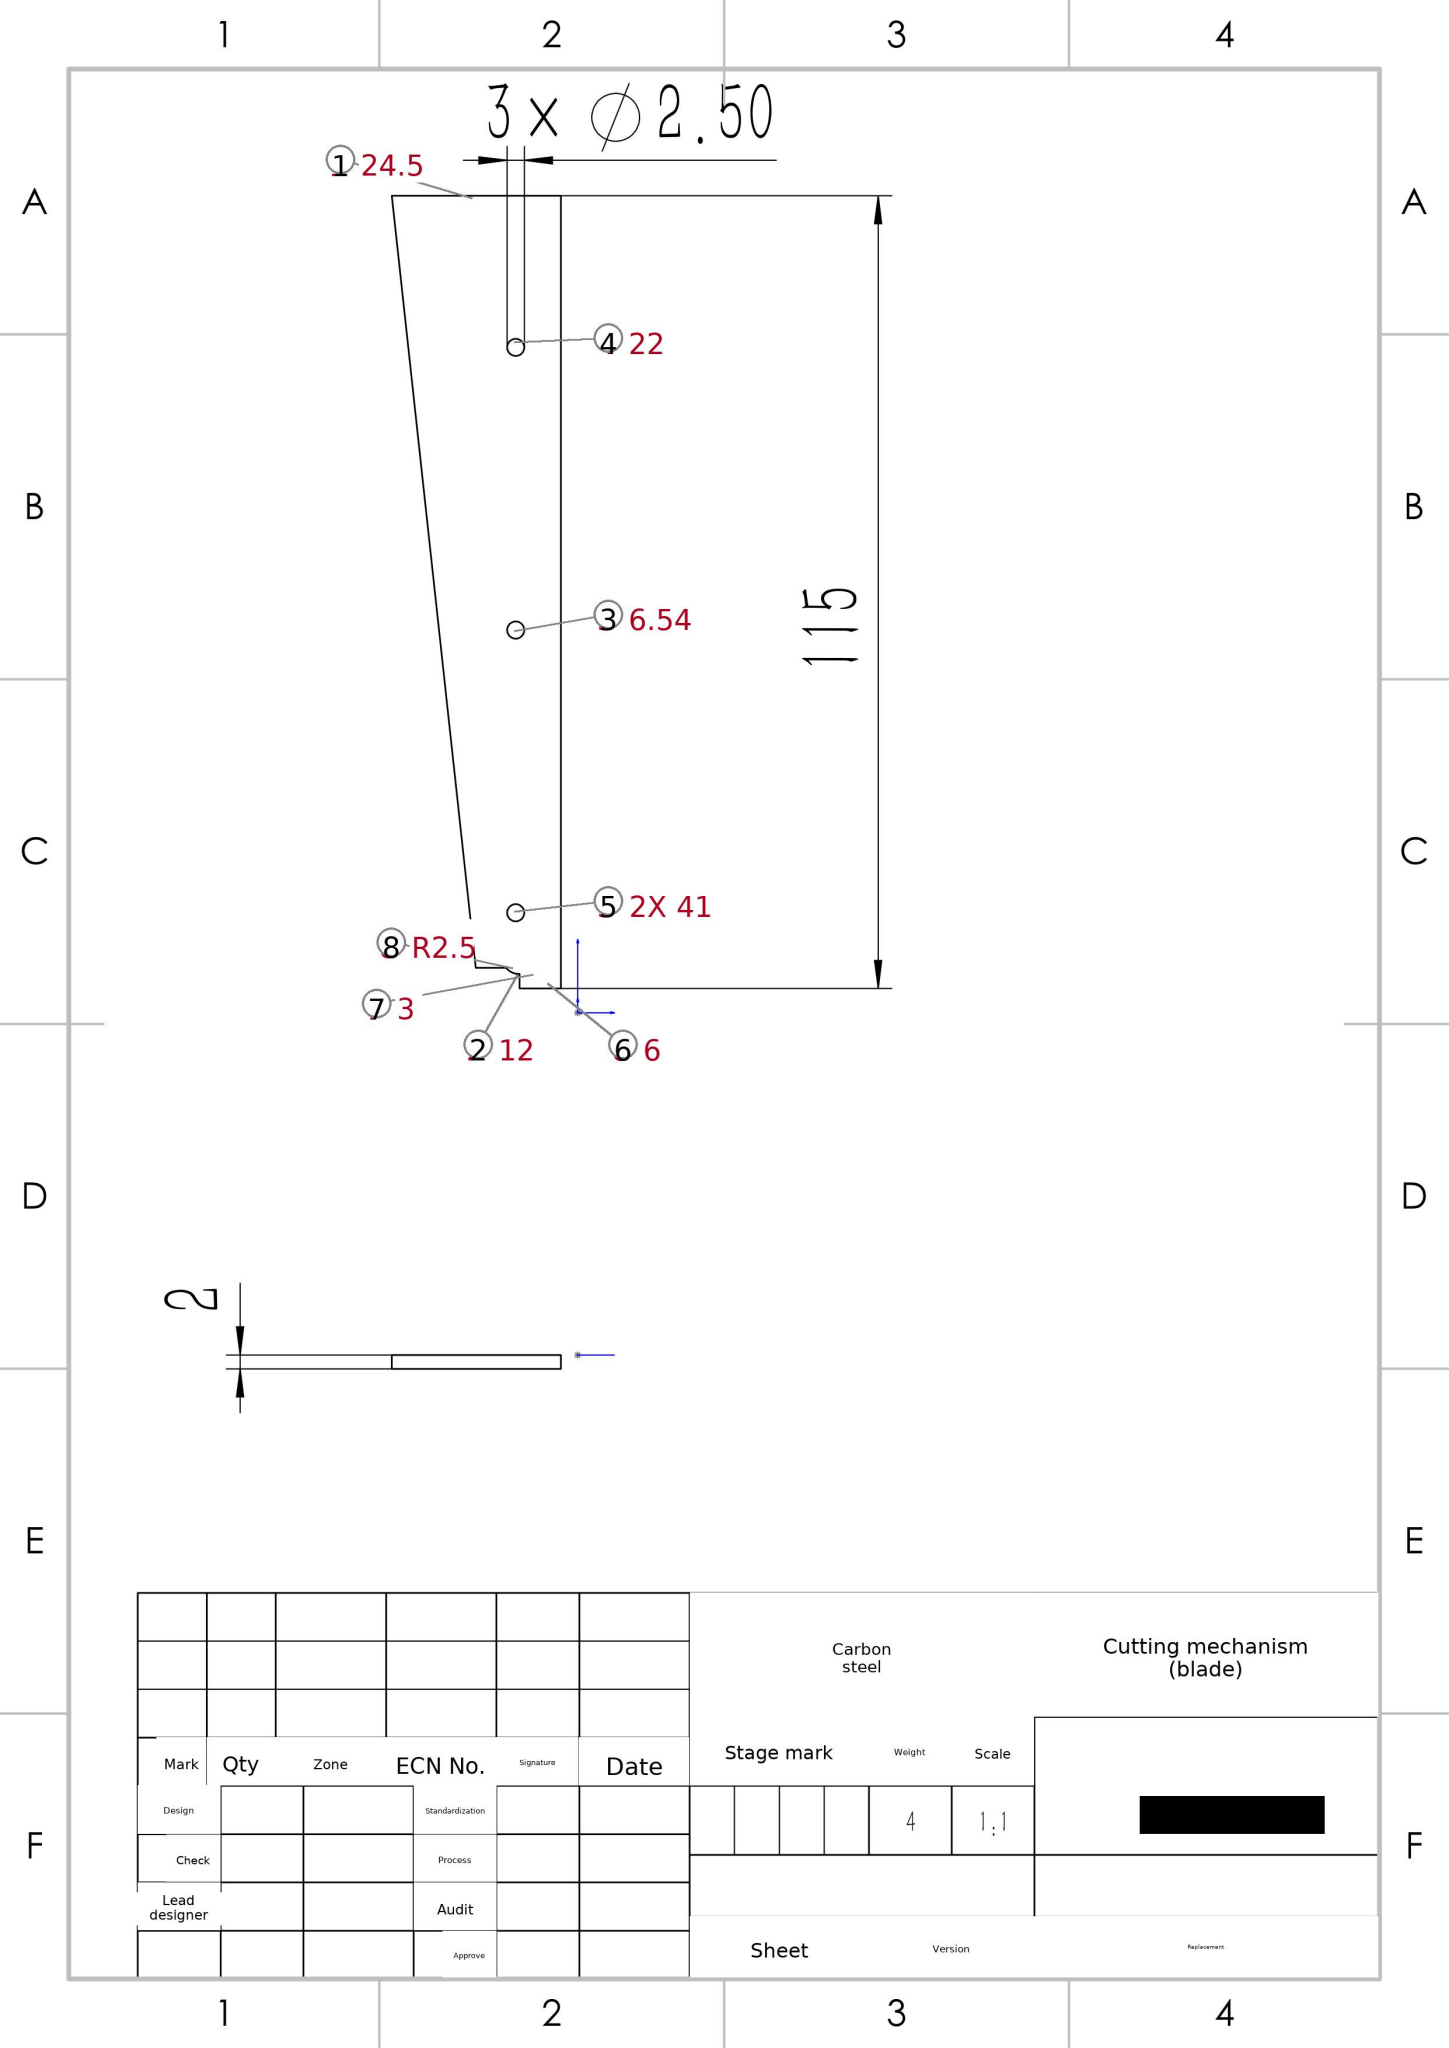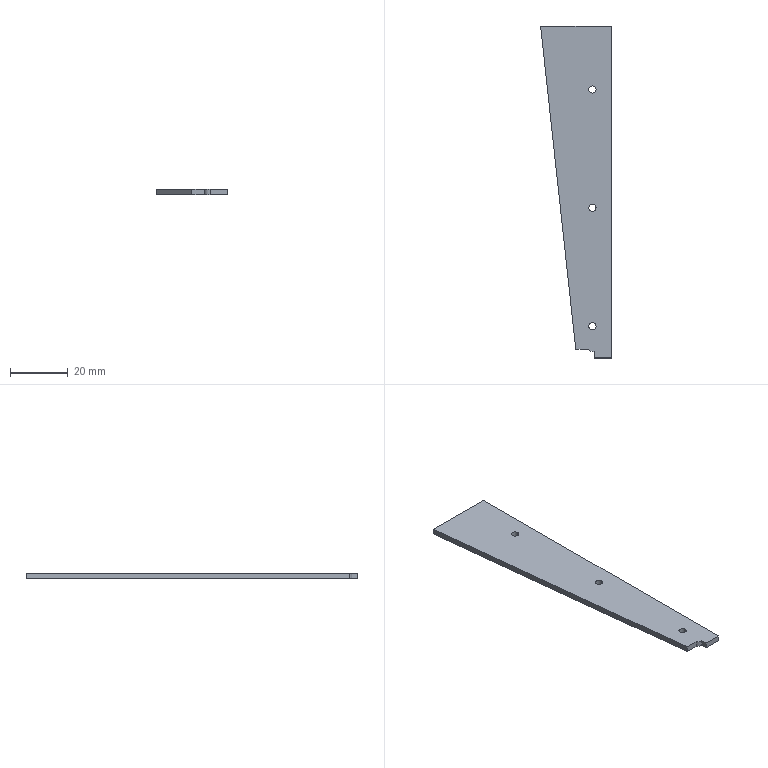Part | SolidWorks | mm | material Carbon steel | 1 solid | 15 faces | box 24.5 x 115 x 2 mm | volume 4133 mm3 | plane 8 | cylinder 7 | commonest cylinder face diameters 2.5 x6 5 x1
STEP:
#1=CARTESIAN_POINT('',(-7.75,96.5,2.));
#2=VERTEX_POINT('',#1);
#3=CARTESIAN_POINT('',(-7.75,96.5,0.));
#4=VERTEX_POINT('',#3);
#5=CARTESIAN_POINT('',(-7.75,96.5,2.));
#6=DIRECTION('',(0.,0.,-1.));
#7=VECTOR('',#6,1000.);
#8=LINE('',#5,#7);
#9=EDGE_CURVE('',#2,#4,#8,.T.);
#10=ORIENTED_EDGE('',*,*,#9,.F.);
#11=CARTESIAN_POINT('',(-10.25,96.5,2.));
#12=VERTEX_POINT('',#11);
#13=CARTESIAN_POINT('',(-9.,96.5,2.));
#14=DIRECTION('',(0.,0.,1.));
#15=DIRECTION('',(1.,0.,0.));
#16=AXIS2_PLACEMENT_3D('',#13,#14,#15);
#17=CIRCLE('',#16,1.25);
#18=EDGE_CURVE('',#2,#12,#17,.T.);
#19=ORIENTED_EDGE('',*,*,#18,.T.);
#20=CARTESIAN_POINT('',(-10.25,96.5,0.));
#21=VERTEX_POINT('',#20);
#22=CARTESIAN_POINT('',(-10.25,96.5,2.));
#23=DIRECTION('',(0.,0.,-1.));
#24=VECTOR('',#23,1000.);
#25=LINE('',#22,#24);
#26=EDGE_CURVE('',#12,#21,#25,.T.);
#27=ORIENTED_EDGE('',*,*,#26,.T.);
#28=CARTESIAN_POINT('',(-9.,96.5,0.));
#29=DIRECTION('',(0.,0.,1.));
#30=DIRECTION('',(1.,0.,0.));
#31=AXIS2_PLACEMENT_3D('',#28,#29,#30);
#32=CIRCLE('',#31,1.25);
#33=EDGE_CURVE('',#4,#21,#32,.T.);
#34=ORIENTED_EDGE('',*,*,#33,.F.);
#35=EDGE_LOOP('',(#10,#19,#27,#34));
#36=FACE_OUTER_BOUND('',#35,.T.);
#37=CARTESIAN_POINT('',(-9.,96.5,2.));
#38=DIRECTION('',(0.,0.,-1.));
#39=DIRECTION('',(-1.,0.,0.));
#40=AXIS2_PLACEMENT_3D('',#37,#38,#39);
#41=CYLINDRICAL_SURFACE('',#40,1.25);
#42=ADVANCED_FACE('',(#36),#41,.F.);
#43=CARTESIAN_POINT('',(-7.75,14.5,2.));
#44=VERTEX_POINT('',#43);
#45=CARTESIAN_POINT('',(-7.75,14.5,0.));
#46=VERTEX_POINT('',#45);
#47=CARTESIAN_POINT('',(-7.75,14.5,2.));
#48=DIRECTION('',(0.,0.,-1.));
#49=VECTOR('',#48,1000.);
#50=LINE('',#47,#49);
#51=EDGE_CURVE('',#44,#46,#50,.T.);
#52=ORIENTED_EDGE('',*,*,#51,.F.);
#53=CARTESIAN_POINT('',(-10.25,14.5,2.));
#54=VERTEX_POINT('',#53);
#55=CARTESIAN_POINT('',(-9.,14.5,2.));
#56=DIRECTION('',(0.,0.,1.));
#57=DIRECTION('',(1.,0.,0.));
#58=AXIS2_PLACEMENT_3D('',#55,#56,#57);
#59=CIRCLE('',#58,1.25);
#60=EDGE_CURVE('',#44,#54,#59,.T.);
#61=ORIENTED_EDGE('',*,*,#60,.T.);
#62=CARTESIAN_POINT('',(-10.25,14.5,0.));
#63=VERTEX_POINT('',#62);
#64=CARTESIAN_POINT('',(-10.25,14.5,2.));
#65=DIRECTION('',(0.,0.,-1.));
#66=VECTOR('',#65,1000.);
#67=LINE('',#64,#66);
#68=EDGE_CURVE('',#54,#63,#67,.T.);
#69=ORIENTED_EDGE('',*,*,#68,.T.);
#70=CARTESIAN_POINT('',(-9.,14.5,0.));
#71=DIRECTION('',(0.,0.,1.));
#72=DIRECTION('',(1.,0.,0.));
#73=AXIS2_PLACEMENT_3D('',#70,#71,#72);
#74=CIRCLE('',#73,1.25);
#75=EDGE_CURVE('',#46,#63,#74,.T.);
#76=ORIENTED_EDGE('',*,*,#75,.F.);
#77=EDGE_LOOP('',(#52,#61,#69,#76));
#78=FACE_OUTER_BOUND('',#77,.T.);
#79=CARTESIAN_POINT('',(-9.,14.5,2.));
#80=DIRECTION('',(0.,0.,-1.));
#81=DIRECTION('',(-1.,0.,0.));
#82=AXIS2_PLACEMENT_3D('',#79,#80,#81);
#83=CYLINDRICAL_SURFACE('',#82,1.25);
#84=ADVANCED_FACE('',(#78),#83,.F.);
#85=CARTESIAN_POINT('',(-7.75,55.5,2.));
#86=VERTEX_POINT('',#85);
#87=CARTESIAN_POINT('',(-7.75,55.5,0.));
#88=VERTEX_POINT('',#87);
#89=CARTESIAN_POINT('',(-7.75,55.5,2.));
#90=DIRECTION('',(0.,0.,-1.));
#91=VECTOR('',#90,1000.);
#92=LINE('',#89,#91);
#93=EDGE_CURVE('',#86,#88,#92,.T.);
#94=ORIENTED_EDGE('',*,*,#93,.F.);
#95=CARTESIAN_POINT('',(-10.25,55.5,2.));
#96=VERTEX_POINT('',#95);
#97=CARTESIAN_POINT('',(-9.,55.5,2.));
#98=DIRECTION('',(0.,0.,1.));
#99=DIRECTION('',(1.,0.,0.));
#100=AXIS2_PLACEMENT_3D('',#97,#98,#99);
#101=CIRCLE('',#100,1.25);
#102=EDGE_CURVE('',#86,#96,#101,.T.);
#103=ORIENTED_EDGE('',*,*,#102,.T.);
#104=CARTESIAN_POINT('',(-10.25,55.5,0.));
#105=VERTEX_POINT('',#104);
#106=CARTESIAN_POINT('',(-10.25,55.5,2.));
#107=DIRECTION('',(0.,0.,-1.));
#108=VECTOR('',#107,1000.);
#109=LINE('',#106,#108);
#110=EDGE_CURVE('',#96,#105,#109,.T.);
#111=ORIENTED_EDGE('',*,*,#110,.T.);
#112=CARTESIAN_POINT('',(-9.,55.5,0.));
#113=DIRECTION('',(0.,0.,1.));
#114=DIRECTION('',(1.,0.,0.));
#115=AXIS2_PLACEMENT_3D('',#112,#113,#114);
#116=CIRCLE('',#115,1.25);
#117=EDGE_CURVE('',#88,#105,#116,.T.);
#118=ORIENTED_EDGE('',*,*,#117,.F.);
#119=EDGE_LOOP('',(#94,#103,#111,#118));
#120=FACE_OUTER_BOUND('',#119,.T.);
#121=CARTESIAN_POINT('',(-9.,55.5,2.));
#122=DIRECTION('',(0.,0.,-1.));
#123=DIRECTION('',(-1.,0.,0.));
#124=AXIS2_PLACEMENT_3D('',#121,#122,#123);
#125=CYLINDRICAL_SURFACE('',#124,1.25);
#126=ADVANCED_FACE('',(#120),#125,.F.);
#127=CARTESIAN_POINT('',(-8.46,5.616,0.));
#128=VERTEX_POINT('',#127);
#129=CARTESIAN_POINT('',(-8.46,3.5,0.));
#130=VERTEX_POINT('',#129);
#131=CARTESIAN_POINT('',(-8.46,0.,0.));
#132=DIRECTION('',(-0.,-1.,0.));
#133=VECTOR('',#132,1000.);
#134=LINE('',#131,#133);
#135=EDGE_CURVE('',#128,#130,#134,.T.);
#136=ORIENTED_EDGE('',*,*,#135,.T.);
#137=CARTESIAN_POINT('',(-8.46,3.5,2.));
#138=VERTEX_POINT('',#137);
#139=CARTESIAN_POINT('',(-8.46,3.5,2.));
#140=DIRECTION('',(0.,0.,-1.));
#141=VECTOR('',#140,1000.);
#142=LINE('',#139,#141);
#143=EDGE_CURVE('',#138,#130,#142,.T.);
#144=ORIENTED_EDGE('',*,*,#143,.F.);
#145=CARTESIAN_POINT('',(-8.46,5.616,2.));
#146=VERTEX_POINT('',#145);
#147=CARTESIAN_POINT('',(-8.46,0.,2.));
#148=DIRECTION('',(-0.,-1.,0.));
#149=VECTOR('',#148,1000.);
#150=LINE('',#147,#149);
#151=EDGE_CURVE('',#146,#138,#150,.T.);
#152=ORIENTED_EDGE('',*,*,#151,.F.);
#153=CARTESIAN_POINT('',(-8.46,5.616,2.));
#154=DIRECTION('',(0.,0.,-1.));
#155=VECTOR('',#154,1000.);
#156=LINE('',#153,#155);
#157=EDGE_CURVE('',#146,#128,#156,.T.);
#158=ORIENTED_EDGE('',*,*,#157,.T.);
#159=EDGE_LOOP('',(#136,#144,#152,#158));
#160=FACE_OUTER_BOUND('',#159,.T.);
#161=CARTESIAN_POINT('',(-8.46,0.,2.));
#162=DIRECTION('',(1.,-0.,0.));
#163=DIRECTION('',(-0.,-1.,0.));
#164=AXIS2_PLACEMENT_3D('',#161,#162,#163);
#165=PLANE('',#164);
#166=ADVANCED_FACE('',(#160),#165,.F.);
#167=CARTESIAN_POINT('',(-14.786,6.5,0.));
#168=VERTEX_POINT('',#167);
#169=CARTESIAN_POINT('',(-10.394,6.5,0.));
#170=VERTEX_POINT('',#169);
#171=CARTESIAN_POINT('',(0.,6.5,0.));
#172=DIRECTION('',(1.,0.,0.));
#173=VECTOR('',#172,1000.);
#174=LINE('',#171,#173);
#175=EDGE_CURVE('',#168,#170,#174,.T.);
#176=ORIENTED_EDGE('',*,*,#175,.T.);
#177=CARTESIAN_POINT('',(-10.394,6.5,2.));
#178=VERTEX_POINT('',#177);
#179=CARTESIAN_POINT('',(-10.394,6.5,2.));
#180=DIRECTION('',(0.,0.,-1.));
#181=VECTOR('',#180,1000.);
#182=LINE('',#179,#181);
#183=EDGE_CURVE('',#178,#170,#182,.T.);
#184=ORIENTED_EDGE('',*,*,#183,.F.);
#185=CARTESIAN_POINT('',(-14.786,6.5,2.));
#186=VERTEX_POINT('',#185);
#187=CARTESIAN_POINT('',(0.,6.5,2.));
#188=DIRECTION('',(1.,0.,0.));
#189=VECTOR('',#188,1000.);
#190=LINE('',#187,#189);
#191=EDGE_CURVE('',#186,#178,#190,.T.);
#192=ORIENTED_EDGE('',*,*,#191,.F.);
#193=CARTESIAN_POINT('',(-14.786,6.5,2.));
#194=DIRECTION('',(0.,0.,-1.));
#195=VECTOR('',#194,1000.);
#196=LINE('',#193,#195);
#197=EDGE_CURVE('',#186,#168,#196,.T.);
#198=ORIENTED_EDGE('',*,*,#197,.T.);
#199=EDGE_LOOP('',(#176,#184,#192,#198));
#200=FACE_OUTER_BOUND('',#199,.T.);
#201=CARTESIAN_POINT('',(0.,6.5,2.));
#202=DIRECTION('',(0.,1.,0.));
#203=DIRECTION('',(1.,0.,0.));
#204=AXIS2_PLACEMENT_3D('',#201,#202,#203);
#205=PLANE('',#204);
#206=ADVANCED_FACE('',(#200),#205,.F.);
#207=CARTESIAN_POINT('',(-8.486,8.116,0.));
#208=DIRECTION('',(0.,0.,1.));
#209=DIRECTION('',(1.,0.,0.));
#210=AXIS2_PLACEMENT_3D('',#207,#208,#209);
#211=CIRCLE('',#210,2.5);
#212=EDGE_CURVE('',#170,#128,#211,.T.);
#213=ORIENTED_EDGE('',*,*,#212,.T.);
#214=ORIENTED_EDGE('',*,*,#157,.F.);
#215=CARTESIAN_POINT('',(-8.486,8.116,2.));
#216=DIRECTION('',(0.,0.,1.));
#217=DIRECTION('',(1.,0.,0.));
#218=AXIS2_PLACEMENT_3D('',#215,#216,#217);
#219=CIRCLE('',#218,2.5);
#220=EDGE_CURVE('',#178,#146,#219,.T.);
#221=ORIENTED_EDGE('',*,*,#220,.F.);
#222=ORIENTED_EDGE('',*,*,#183,.T.);
#223=EDGE_LOOP('',(#213,#214,#221,#222));
#224=FACE_OUTER_BOUND('',#223,.T.);
#225=CARTESIAN_POINT('',(-8.486,8.116,2.));
#226=DIRECTION('',(0.,0.,-1.));
#227=DIRECTION('',(-1.,0.,0.));
#228=AXIS2_PLACEMENT_3D('',#225,#226,#227);
#229=CYLINDRICAL_SURFACE('',#228,2.5);
#230=ADVANCED_FACE('',(#224),#229,.T.);
#231=CARTESIAN_POINT('',(-2.46,118.5,0.));
#232=VERTEX_POINT('',#231);
#233=CARTESIAN_POINT('',(-2.46,3.5,0.));
#234=VERTEX_POINT('',#233);
#235=CARTESIAN_POINT('',(-2.46,118.5,0.));
#236=DIRECTION('',(0.,-1.,0.));
#237=VECTOR('',#236,1000.);
#238=LINE('',#235,#237);
#239=EDGE_CURVE('',#232,#234,#238,.T.);
#240=ORIENTED_EDGE('',*,*,#239,.F.);
#241=CARTESIAN_POINT('',(-2.46,118.5,2.));
#242=VERTEX_POINT('',#241);
#243=CARTESIAN_POINT('',(-2.46,118.5,2.));
#244=DIRECTION('',(0.,0.,-1.));
#245=VECTOR('',#244,1000.);
#246=LINE('',#243,#245);
#247=EDGE_CURVE('',#242,#232,#246,.T.);
#248=ORIENTED_EDGE('',*,*,#247,.F.);
#249=CARTESIAN_POINT('',(-2.46,3.5,2.));
#250=VERTEX_POINT('',#249);
#251=CARTESIAN_POINT('',(-2.46,118.5,2.));
#252=DIRECTION('',(0.,-1.,0.));
#253=VECTOR('',#252,1000.);
#254=LINE('',#251,#253);
#255=EDGE_CURVE('',#242,#250,#254,.T.);
#256=ORIENTED_EDGE('',*,*,#255,.T.);
#257=CARTESIAN_POINT('',(-2.46,3.5,2.));
#258=DIRECTION('',(0.,0.,-1.));
#259=VECTOR('',#258,1000.);
#260=LINE('',#257,#259);
#261=EDGE_CURVE('',#250,#234,#260,.T.);
#262=ORIENTED_EDGE('',*,*,#261,.T.);
#263=EDGE_LOOP('',(#240,#248,#256,#262));
#264=FACE_OUTER_BOUND('',#263,.T.);
#265=CARTESIAN_POINT('',(-2.46,118.5,2.));
#266=DIRECTION('',(1.,0.,0.));
#267=DIRECTION('',(-0.,1.,0.));
#268=AXIS2_PLACEMENT_3D('',#265,#266,#267);
#269=PLANE('',#268);
#270=ADVANCED_FACE('',(#264),#269,.T.);
#271=CARTESIAN_POINT('',(-14.46,3.5,2.));
#272=DIRECTION('',(1.,0.,0.));
#273=VECTOR('',#272,1000.);
#274=LINE('',#271,#273);
#275=EDGE_CURVE('',#138,#250,#274,.T.);
#276=ORIENTED_EDGE('',*,*,#275,.F.);
#277=ORIENTED_EDGE('',*,*,#143,.T.);
#278=CARTESIAN_POINT('',(-14.46,3.5,0.));
#279=DIRECTION('',(1.,0.,0.));
#280=VECTOR('',#279,1000.);
#281=LINE('',#278,#280);
#282=EDGE_CURVE('',#130,#234,#281,.T.);
#283=ORIENTED_EDGE('',*,*,#282,.T.);
#284=ORIENTED_EDGE('',*,*,#261,.F.);
#285=EDGE_LOOP('',(#276,#277,#283,#284));
#286=FACE_OUTER_BOUND('',#285,.T.);
#287=CARTESIAN_POINT('',(-14.46,3.5,2.));
#288=DIRECTION('',(-0.,1.,0.));
#289=DIRECTION('',(1.,0.,0.));
#290=AXIS2_PLACEMENT_3D('',#287,#288,#289);
#291=PLANE('',#290);
#292=ADVANCED_FACE('',(#286),#291,.F.);
#293=ORIENTED_EDGE('',*,*,#197,.F.);
#294=CARTESIAN_POINT('',(-26.96,118.5,2.));
#295=VERTEX_POINT('',#294);
#296=CARTESIAN_POINT('',(-14.46,3.5,2.));
#297=DIRECTION('',(-0.1081,0.9941,0.));
#298=VECTOR('',#297,1000.);
#299=LINE('',#296,#298);
#300=EDGE_CURVE('',#186,#295,#299,.T.);
#301=ORIENTED_EDGE('',*,*,#300,.T.);
#302=CARTESIAN_POINT('',(-26.96,118.5,0.));
#303=VERTEX_POINT('',#302);
#304=CARTESIAN_POINT('',(-26.96,118.5,2.));
#305=DIRECTION('',(0.,0.,-1.));
#306=VECTOR('',#305,1000.);
#307=LINE('',#304,#306);
#308=EDGE_CURVE('',#295,#303,#307,.T.);
#309=ORIENTED_EDGE('',*,*,#308,.T.);
#310=CARTESIAN_POINT('',(-14.46,3.5,0.));
#311=DIRECTION('',(-0.1081,0.9941,0.));
#312=VECTOR('',#311,1000.);
#313=LINE('',#310,#312);
#314=EDGE_CURVE('',#168,#303,#313,.T.);
#315=ORIENTED_EDGE('',*,*,#314,.F.);
#316=EDGE_LOOP('',(#293,#301,#309,#315));
#317=FACE_OUTER_BOUND('',#316,.T.);
#318=CARTESIAN_POINT('',(-14.46,3.5,2.));
#319=DIRECTION('',(-0.9941,-0.1081,0.));
#320=DIRECTION('',(-0.1081,0.9941,0.));
#321=AXIS2_PLACEMENT_3D('',#318,#319,#320);
#322=PLANE('',#321);
#323=ADVANCED_FACE('',(#317),#322,.T.);
#324=CARTESIAN_POINT('',(-26.96,118.5,0.));
#325=DIRECTION('',(1.,-0.,0.));
#326=VECTOR('',#325,1000.);
#327=LINE('',#324,#326);
#328=EDGE_CURVE('',#303,#232,#327,.T.);
#329=ORIENTED_EDGE('',*,*,#328,.F.);
#330=ORIENTED_EDGE('',*,*,#308,.F.);
#331=CARTESIAN_POINT('',(-26.96,118.5,2.));
#332=DIRECTION('',(1.,-0.,0.));
#333=VECTOR('',#332,1000.);
#334=LINE('',#331,#333);
#335=EDGE_CURVE('',#295,#242,#334,.T.);
#336=ORIENTED_EDGE('',*,*,#335,.T.);
#337=ORIENTED_EDGE('',*,*,#247,.T.);
#338=EDGE_LOOP('',(#329,#330,#336,#337));
#339=FACE_OUTER_BOUND('',#338,.T.);
#340=CARTESIAN_POINT('',(-26.96,118.5,2.));
#341=DIRECTION('',(0.,1.,0.));
#342=DIRECTION('',(1.,-0.,0.));
#343=AXIS2_PLACEMENT_3D('',#340,#341,#342);
#344=PLANE('',#343);
#345=ADVANCED_FACE('',(#339),#344,.T.);
#346=CARTESIAN_POINT('',(-9.,96.5,0.));
#347=DIRECTION('',(0.,0.,1.));
#348=DIRECTION('',(1.,0.,0.));
#349=AXIS2_PLACEMENT_3D('',#346,#347,#348);
#350=CIRCLE('',#349,1.25);
#351=EDGE_CURVE('',#21,#4,#350,.T.);
#352=ORIENTED_EDGE('',*,*,#351,.T.);
#353=ORIENTED_EDGE('',*,*,#33,.T.);
#354=EDGE_LOOP('',(#352,#353));
#355=FACE_BOUND('',#354,.T.);
#356=CARTESIAN_POINT('',(-9.,55.5,0.));
#357=DIRECTION('',(0.,0.,1.));
#358=DIRECTION('',(1.,0.,0.));
#359=AXIS2_PLACEMENT_3D('',#356,#357,#358);
#360=CIRCLE('',#359,1.25);
#361=EDGE_CURVE('',#105,#88,#360,.T.);
#362=ORIENTED_EDGE('',*,*,#361,.T.);
#363=ORIENTED_EDGE('',*,*,#117,.T.);
#364=EDGE_LOOP('',(#362,#363));
#365=FACE_BOUND('',#364,.T.);
#366=CARTESIAN_POINT('',(-9.,14.5,0.));
#367=DIRECTION('',(0.,0.,1.));
#368=DIRECTION('',(1.,0.,0.));
#369=AXIS2_PLACEMENT_3D('',#366,#367,#368);
#370=CIRCLE('',#369,1.25);
#371=EDGE_CURVE('',#63,#46,#370,.T.);
#372=ORIENTED_EDGE('',*,*,#371,.T.);
#373=ORIENTED_EDGE('',*,*,#75,.T.);
#374=EDGE_LOOP('',(#372,#373));
#375=FACE_BOUND('',#374,.T.);
#376=ORIENTED_EDGE('',*,*,#175,.F.);
#377=ORIENTED_EDGE('',*,*,#314,.T.);
#378=ORIENTED_EDGE('',*,*,#328,.T.);
#379=ORIENTED_EDGE('',*,*,#239,.T.);
#380=ORIENTED_EDGE('',*,*,#282,.F.);
#381=ORIENTED_EDGE('',*,*,#135,.F.);
#382=ORIENTED_EDGE('',*,*,#212,.F.);
#383=EDGE_LOOP('',(#376,#377,#378,#379,#380,#381,#382));
#384=FACE_OUTER_BOUND('',#383,.T.);
#385=CARTESIAN_POINT('',(0.,0.,0.));
#386=DIRECTION('',(0.,0.,-1.));
#387=DIRECTION('',(0.,-1.,0.));
#388=AXIS2_PLACEMENT_3D('',#385,#386,#387);
#389=PLANE('',#388);
#390=ADVANCED_FACE('',(#355,#365,#375,#384),#389,.T.);
#391=CARTESIAN_POINT('',(-9.,96.5,2.));
#392=DIRECTION('',(0.,0.,1.));
#393=DIRECTION('',(1.,0.,0.));
#394=AXIS2_PLACEMENT_3D('',#391,#392,#393);
#395=CIRCLE('',#394,1.25);
#396=EDGE_CURVE('',#12,#2,#395,.T.);
#397=ORIENTED_EDGE('',*,*,#396,.F.);
#398=ORIENTED_EDGE('',*,*,#18,.F.);
#399=EDGE_LOOP('',(#397,#398));
#400=FACE_BOUND('',#399,.T.);
#401=CARTESIAN_POINT('',(-9.,55.5,2.));
#402=DIRECTION('',(0.,0.,1.));
#403=DIRECTION('',(1.,0.,0.));
#404=AXIS2_PLACEMENT_3D('',#401,#402,#403);
#405=CIRCLE('',#404,1.25);
#406=EDGE_CURVE('',#96,#86,#405,.T.);
#407=ORIENTED_EDGE('',*,*,#406,.F.);
#408=ORIENTED_EDGE('',*,*,#102,.F.);
#409=EDGE_LOOP('',(#407,#408));
#410=FACE_BOUND('',#409,.T.);
#411=CARTESIAN_POINT('',(-9.,14.5,2.));
#412=DIRECTION('',(0.,0.,1.));
#413=DIRECTION('',(1.,0.,0.));
#414=AXIS2_PLACEMENT_3D('',#411,#412,#413);
#415=CIRCLE('',#414,1.25);
#416=EDGE_CURVE('',#54,#44,#415,.T.);
#417=ORIENTED_EDGE('',*,*,#416,.F.);
#418=ORIENTED_EDGE('',*,*,#60,.F.);
#419=EDGE_LOOP('',(#417,#418));
#420=FACE_BOUND('',#419,.T.);
#421=ORIENTED_EDGE('',*,*,#300,.F.);
#422=ORIENTED_EDGE('',*,*,#191,.T.);
#423=ORIENTED_EDGE('',*,*,#220,.T.);
#424=ORIENTED_EDGE('',*,*,#151,.T.);
#425=ORIENTED_EDGE('',*,*,#275,.T.);
#426=ORIENTED_EDGE('',*,*,#255,.F.);
#427=ORIENTED_EDGE('',*,*,#335,.F.);
#428=EDGE_LOOP('',(#421,#422,#423,#424,#425,#426,#427));
#429=FACE_OUTER_BOUND('',#428,.T.);
#430=CARTESIAN_POINT('',(0.,0.,2.));
#431=DIRECTION('',(0.,0.,-1.));
#432=DIRECTION('',(0.,-1.,0.));
#433=AXIS2_PLACEMENT_3D('',#430,#431,#432);
#434=PLANE('',#433);
#435=ADVANCED_FACE('',(#400,#410,#420,#429),#434,.F.);
#436=ORIENTED_EDGE('',*,*,#406,.T.);
#437=ORIENTED_EDGE('',*,*,#93,.T.);
#438=ORIENTED_EDGE('',*,*,#361,.F.);
#439=ORIENTED_EDGE('',*,*,#110,.F.);
#440=EDGE_LOOP('',(#436,#437,#438,#439));
#441=FACE_OUTER_BOUND('',#440,.T.);
#442=CARTESIAN_POINT('',(-9.,55.5,2.));
#443=DIRECTION('',(0.,0.,-1.));
#444=DIRECTION('',(-1.,0.,0.));
#445=AXIS2_PLACEMENT_3D('',#442,#443,#444);
#446=CYLINDRICAL_SURFACE('',#445,1.25);
#447=ADVANCED_FACE('',(#441),#446,.F.);
#448=ORIENTED_EDGE('',*,*,#416,.T.);
#449=ORIENTED_EDGE('',*,*,#51,.T.);
#450=ORIENTED_EDGE('',*,*,#371,.F.);
#451=ORIENTED_EDGE('',*,*,#68,.F.);
#452=EDGE_LOOP('',(#448,#449,#450,#451));
#453=FACE_OUTER_BOUND('',#452,.T.);
#454=CARTESIAN_POINT('',(-9.,14.5,2.));
#455=DIRECTION('',(0.,0.,-1.));
#456=DIRECTION('',(-1.,0.,0.));
#457=AXIS2_PLACEMENT_3D('',#454,#455,#456);
#458=CYLINDRICAL_SURFACE('',#457,1.25);
#459=ADVANCED_FACE('',(#453),#458,.F.);
#460=ORIENTED_EDGE('',*,*,#396,.T.);
#461=ORIENTED_EDGE('',*,*,#9,.T.);
#462=ORIENTED_EDGE('',*,*,#351,.F.);
#463=ORIENTED_EDGE('',*,*,#26,.F.);
#464=EDGE_LOOP('',(#460,#461,#462,#463));
#465=FACE_OUTER_BOUND('',#464,.T.);
#466=CARTESIAN_POINT('',(-9.,96.5,2.));
#467=DIRECTION('',(0.,0.,-1.));
#468=DIRECTION('',(-1.,0.,0.));
#469=AXIS2_PLACEMENT_3D('',#466,#467,#468);
#470=CYLINDRICAL_SURFACE('',#469,1.25);
#471=ADVANCED_FACE('',(#465),#470,.F.);
#472=CLOSED_SHELL('',(#42,#84,#126,#166,#206,#230,#270,#292,#323,#345,#390,#435,#447,#459,#471));
#473=MANIFOLD_SOLID_BREP('',#472);
#474=CARTESIAN_POINT('',(0.,0.,0.));
#475=DIRECTION('',(0.,0.,1.));
#476=DIRECTION('',(1.,0.,0.));
#477=AXIS2_PLACEMENT_3D('',#474,#475,#476);
#478=(LENGTH_UNIT()NAMED_UNIT(*)SI_UNIT(.MILLI.,.METRE.));
#479=UNCERTAINTY_MEASURE_WITH_UNIT(LENGTH_MEASURE(0.00001),#478,'','');
#480=(NAMED_UNIT(*)PLANE_ANGLE_UNIT()SI_UNIT($,.RADIAN.));
#481=(NAMED_UNIT(*)SI_UNIT($,.STERADIAN.)SOLID_ANGLE_UNIT());
#482=(GEOMETRIC_REPRESENTATION_CONTEXT(3)GLOBAL_UNCERTAINTY_ASSIGNED_CONTEXT((#479))GLOBAL_UNIT_ASSIGNED_CONTEXT((#478,#480,#481))REPRESENTATION_CONTEXT('',''));
#483=ADVANCED_BREP_SHAPE_REPRESENTATION('',(#473,#477),#482);